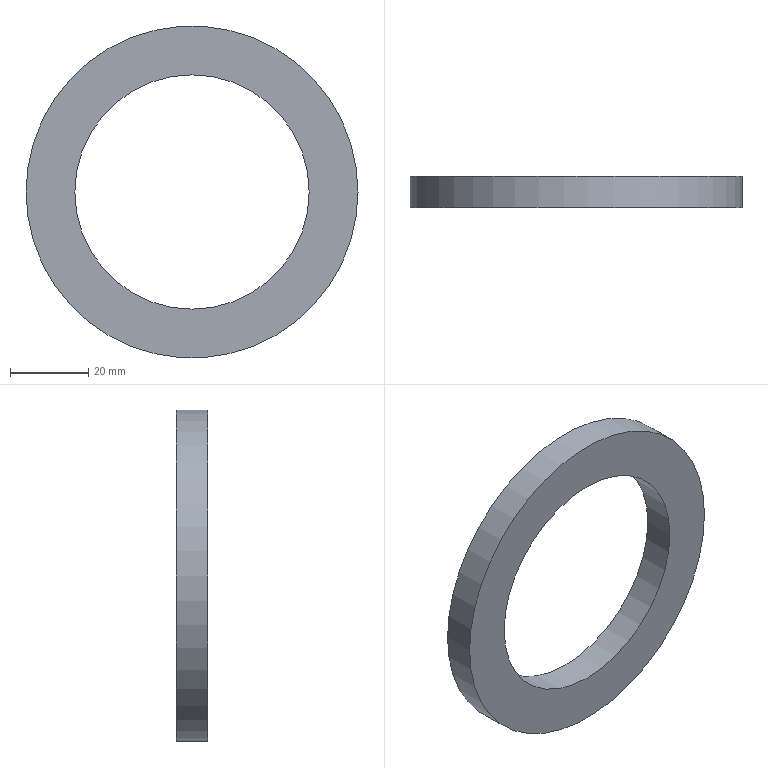Component | NX | OIL_SEAL_85X60X8_2 | 1 solid | 4 faces | box 85 x 8 x 85 mm | volume 22777 mm3 | cylinder 2 | plane 2 | commonest cylinder face diameters 85 x1 60 x1
STEP:
#1=CARTESIAN_POINT('',(0.,0.,0.));
#2=DIRECTION('',(0.,0.,1.));
#3=DIRECTION('',(1.,0.,0.));
#4=AXIS2_PLACEMENT_3D('',#1,#2,#3);
#5=CARTESIAN_POINT('',(47.5,-94.,265.5));
#6=VERTEX_POINT('',#5);
#7=CARTESIAN_POINT('',(5.,-94.,265.5));
#8=DIRECTION('',(0.,-1.,0.));
#9=DIRECTION('',(1.,0.,0.));
#10=AXIS2_PLACEMENT_3D('',#7,#8,#9);
#11=CIRCLE('',#10,42.5);
#12=CARTESIAN_POINT('',(5.,-94.,265.5));
#13=DIRECTION('',(0.,1.,0.));
#14=DIRECTION('',(-1.,0.,-0.));
#15=AXIS2_PLACEMENT_3D('',#12,#13,#14);
#16=CYLINDRICAL_SURFACE('',#15,42.5);
#17=CARTESIAN_POINT('',(9.425,0.));
#18=DIRECTION('',(-1.,0.));
#19=VECTOR('',#18,1.);
#20=LINE('',#17,#19);
#21=(GEOMETRIC_REPRESENTATION_CONTEXT(2)PARAMETRIC_REPRESENTATION_CONTEXT()REPRESENTATION_CONTEXT('',''));
#22=DEFINITIONAL_REPRESENTATION('',(#20),#21);
#23=PCURVE('',#16,#22);
#24=CARTESIAN_POINT('',(5.,-94.,265.5));
#25=DIRECTION('',(0.,-1.,0.));
#26=DIRECTION('',(1.,0.,0.));
#27=AXIS2_PLACEMENT_3D('',#24,#25,#26);
#28=PLANE('',#27);
#29=CARTESIAN_POINT('',(0.,0.));
#30=DIRECTION('',(1.,-0.));
#31=AXIS2_PLACEMENT_2D('',#29,#30);
#32=CIRCLE('',#31,42.5);
#33=(GEOMETRIC_REPRESENTATION_CONTEXT(2)PARAMETRIC_REPRESENTATION_CONTEXT()REPRESENTATION_CONTEXT('',''));
#34=DEFINITIONAL_REPRESENTATION('',(#32),#33);
#35=PCURVE('',#28,#34);
#36=SURFACE_CURVE('',#11,(#23,#35),.PCURVE_S1.);
#37=EDGE_CURVE('',#6,#6,#36,.T.);
#38=ORIENTED_EDGE('',*,*,#37,.F.);
#39=CARTESIAN_POINT('',(47.5,-86.,265.5));
#40=VERTEX_POINT('',#39);
#41=CARTESIAN_POINT('',(47.5,-94.,265.5));
#42=CARTESIAN_POINT('',(47.5,-86.,265.5));
#43=B_SPLINE_CURVE_WITH_KNOTS('',1,(#41,#42),.UNSPECIFIED.,.F.,.F.,(2,2),(0.,8.),.PIECEWISE_BEZIER_KNOTS.);
#44=CARTESIAN_POINT('',(9.425,0.));
#45=DIRECTION('',(0.,1.));
#46=VECTOR('',#45,1.);
#47=LINE('',#44,#46);
#48=(GEOMETRIC_REPRESENTATION_CONTEXT(2)PARAMETRIC_REPRESENTATION_CONTEXT()REPRESENTATION_CONTEXT('',''));
#49=DEFINITIONAL_REPRESENTATION('',(#47),#48);
#50=PCURVE('',#16,#49);
#51=CARTESIAN_POINT('',(3.142,0.));
#52=DIRECTION('',(0.,1.));
#53=VECTOR('',#52,1.);
#54=LINE('',#51,#53);
#55=(GEOMETRIC_REPRESENTATION_CONTEXT(2)PARAMETRIC_REPRESENTATION_CONTEXT()REPRESENTATION_CONTEXT('',''));
#56=DEFINITIONAL_REPRESENTATION('',(#54),#55);
#57=PCURVE('',#16,#56);
#58=SEAM_CURVE('',#43,(#50,#57),.PCURVE_S1.);
#59=EDGE_CURVE('',#6,#40,#58,.T.);
#60=ORIENTED_EDGE('',*,*,#59,.T.);
#61=CARTESIAN_POINT('',(5.,-86.,265.5));
#62=DIRECTION('',(0.,-1.,0.));
#63=DIRECTION('',(1.,0.,0.));
#64=AXIS2_PLACEMENT_3D('',#61,#62,#63);
#65=CIRCLE('',#64,42.5);
#66=CARTESIAN_POINT('',(9.425,8.));
#67=DIRECTION('',(-1.,0.));
#68=VECTOR('',#67,1.);
#69=LINE('',#66,#68);
#70=(GEOMETRIC_REPRESENTATION_CONTEXT(2)PARAMETRIC_REPRESENTATION_CONTEXT()REPRESENTATION_CONTEXT('',''));
#71=DEFINITIONAL_REPRESENTATION('',(#69),#70);
#72=PCURVE('',#16,#71);
#73=CARTESIAN_POINT('',(5.,-86.,265.5));
#74=DIRECTION('',(0.,-1.,0.));
#75=DIRECTION('',(1.,0.,0.));
#76=AXIS2_PLACEMENT_3D('',#73,#74,#75);
#77=PLANE('',#76);
#78=CARTESIAN_POINT('',(0.,0.));
#79=DIRECTION('',(1.,-0.));
#80=AXIS2_PLACEMENT_2D('',#78,#79);
#81=CIRCLE('',#80,42.5);
#82=(GEOMETRIC_REPRESENTATION_CONTEXT(2)PARAMETRIC_REPRESENTATION_CONTEXT()REPRESENTATION_CONTEXT('',''));
#83=DEFINITIONAL_REPRESENTATION('',(#81),#82);
#84=PCURVE('',#77,#83);
#85=SURFACE_CURVE('',#65,(#72,#84),.PCURVE_S1.);
#86=EDGE_CURVE('',#40,#40,#85,.T.);
#87=ORIENTED_EDGE('',*,*,#86,.T.);
#88=ORIENTED_EDGE('',*,*,#59,.F.);
#89=EDGE_LOOP('',(#38,#60,#87,#88));
#90=FACE_BOUND('',#89,.T.);
#91=ADVANCED_FACE('',(#90),#16,.T.);
#92=CARTESIAN_POINT('',(35.,-94.,265.5));
#93=VERTEX_POINT('',#92);
#94=CARTESIAN_POINT('',(5.,-94.,265.5));
#95=DIRECTION('',(0.,-1.,0.));
#96=DIRECTION('',(1.,0.,0.));
#97=AXIS2_PLACEMENT_3D('',#94,#95,#96);
#98=CIRCLE('',#97,30.);
#99=CARTESIAN_POINT('',(5.,-94.,265.5));
#100=DIRECTION('',(0.,1.,0.));
#101=DIRECTION('',(-1.,0.,-0.));
#102=AXIS2_PLACEMENT_3D('',#99,#100,#101);
#103=CYLINDRICAL_SURFACE('',#102,30.);
#104=CARTESIAN_POINT('',(9.425,0.));
#105=DIRECTION('',(-1.,0.));
#106=VECTOR('',#105,1.);
#107=LINE('',#104,#106);
#108=(GEOMETRIC_REPRESENTATION_CONTEXT(2)PARAMETRIC_REPRESENTATION_CONTEXT()REPRESENTATION_CONTEXT('',''));
#109=DEFINITIONAL_REPRESENTATION('',(#107),#108);
#110=PCURVE('',#103,#109);
#111=CARTESIAN_POINT('',(0.,0.));
#112=DIRECTION('',(1.,-0.));
#113=AXIS2_PLACEMENT_2D('',#111,#112);
#114=CIRCLE('',#113,30.);
#115=(GEOMETRIC_REPRESENTATION_CONTEXT(2)PARAMETRIC_REPRESENTATION_CONTEXT()REPRESENTATION_CONTEXT('',''));
#116=DEFINITIONAL_REPRESENTATION('',(#114),#115);
#117=PCURVE('',#28,#116);
#118=SURFACE_CURVE('',#98,(#110,#117),.PCURVE_S1.);
#119=EDGE_CURVE('',#93,#93,#118,.T.);
#120=ORIENTED_EDGE('',*,*,#119,.F.);
#121=CARTESIAN_POINT('',(35.,-86.,265.5));
#122=VERTEX_POINT('',#121);
#123=CARTESIAN_POINT('',(35.,-94.,265.5));
#124=CARTESIAN_POINT('',(35.,-86.,265.5));
#125=B_SPLINE_CURVE_WITH_KNOTS('',1,(#123,#124),.UNSPECIFIED.,.F.,.F.,(2,2),(0.,8.),.PIECEWISE_BEZIER_KNOTS.);
#126=CARTESIAN_POINT('',(9.425,0.));
#127=DIRECTION('',(0.,1.));
#128=VECTOR('',#127,1.);
#129=LINE('',#126,#128);
#130=(GEOMETRIC_REPRESENTATION_CONTEXT(2)PARAMETRIC_REPRESENTATION_CONTEXT()REPRESENTATION_CONTEXT('',''));
#131=DEFINITIONAL_REPRESENTATION('',(#129),#130);
#132=PCURVE('',#103,#131);
#133=CARTESIAN_POINT('',(3.142,0.));
#134=DIRECTION('',(0.,1.));
#135=VECTOR('',#134,1.);
#136=LINE('',#133,#135);
#137=(GEOMETRIC_REPRESENTATION_CONTEXT(2)PARAMETRIC_REPRESENTATION_CONTEXT()REPRESENTATION_CONTEXT('',''));
#138=DEFINITIONAL_REPRESENTATION('',(#136),#137);
#139=PCURVE('',#103,#138);
#140=SEAM_CURVE('',#125,(#132,#139),.PCURVE_S1.);
#141=EDGE_CURVE('',#93,#122,#140,.T.);
#142=ORIENTED_EDGE('',*,*,#141,.T.);
#143=CARTESIAN_POINT('',(5.,-86.,265.5));
#144=DIRECTION('',(0.,-1.,0.));
#145=DIRECTION('',(1.,0.,0.));
#146=AXIS2_PLACEMENT_3D('',#143,#144,#145);
#147=CIRCLE('',#146,30.);
#148=CARTESIAN_POINT('',(9.425,8.));
#149=DIRECTION('',(-1.,0.));
#150=VECTOR('',#149,1.);
#151=LINE('',#148,#150);
#152=(GEOMETRIC_REPRESENTATION_CONTEXT(2)PARAMETRIC_REPRESENTATION_CONTEXT()REPRESENTATION_CONTEXT('',''));
#153=DEFINITIONAL_REPRESENTATION('',(#151),#152);
#154=PCURVE('',#103,#153);
#155=CARTESIAN_POINT('',(0.,0.));
#156=DIRECTION('',(1.,-0.));
#157=AXIS2_PLACEMENT_2D('',#155,#156);
#158=CIRCLE('',#157,30.);
#159=(GEOMETRIC_REPRESENTATION_CONTEXT(2)PARAMETRIC_REPRESENTATION_CONTEXT()REPRESENTATION_CONTEXT('',''));
#160=DEFINITIONAL_REPRESENTATION('',(#158),#159);
#161=PCURVE('',#77,#160);
#162=SURFACE_CURVE('',#147,(#154,#161),.PCURVE_S1.);
#163=EDGE_CURVE('',#122,#122,#162,.T.);
#164=ORIENTED_EDGE('',*,*,#163,.T.);
#165=ORIENTED_EDGE('',*,*,#141,.F.);
#166=EDGE_LOOP('',(#120,#142,#164,#165));
#167=FACE_BOUND('',#166,.F.);
#168=ADVANCED_FACE('',(#167),#103,.F.);
#169=ORIENTED_EDGE('',*,*,#37,.T.);
#170=EDGE_LOOP('',(#169));
#171=FACE_BOUND('',#170,.T.);
#172=ORIENTED_EDGE('',*,*,#119,.F.);
#173=EDGE_LOOP('',(#172));
#174=FACE_BOUND('',#173,.T.);
#175=ADVANCED_FACE('',(#171,#174),#28,.T.);
#176=ORIENTED_EDGE('',*,*,#86,.F.);
#177=EDGE_LOOP('',(#176));
#178=FACE_BOUND('',#177,.T.);
#179=ORIENTED_EDGE('',*,*,#163,.T.);
#180=EDGE_LOOP('',(#179));
#181=FACE_BOUND('',#180,.T.);
#182=ADVANCED_FACE('',(#178,#181),#77,.F.);
#183=CLOSED_SHELL('',(#91,#168,#175,#182));
#184=MANIFOLD_SOLID_BREP('',#183);
#185=(LENGTH_UNIT()NAMED_UNIT(*)SI_UNIT(.MILLI.,.METRE.));
#186=UNCERTAINTY_MEASURE_WITH_UNIT(LENGTH_MEASURE(0.00001),#185,'','');
#187=(NAMED_UNIT(*)PLANE_ANGLE_UNIT()SI_UNIT($,.RADIAN.));
#188=(NAMED_UNIT(*)SI_UNIT($,.STERADIAN.)SOLID_ANGLE_UNIT());
#189=(GEOMETRIC_REPRESENTATION_CONTEXT(3)GLOBAL_UNCERTAINTY_ASSIGNED_CONTEXT((#186))GLOBAL_UNIT_ASSIGNED_CONTEXT((#185,#187,#188))REPRESENTATION_CONTEXT('',''));
#190=ADVANCED_BREP_SHAPE_REPRESENTATION('',(#4,#184),#189);